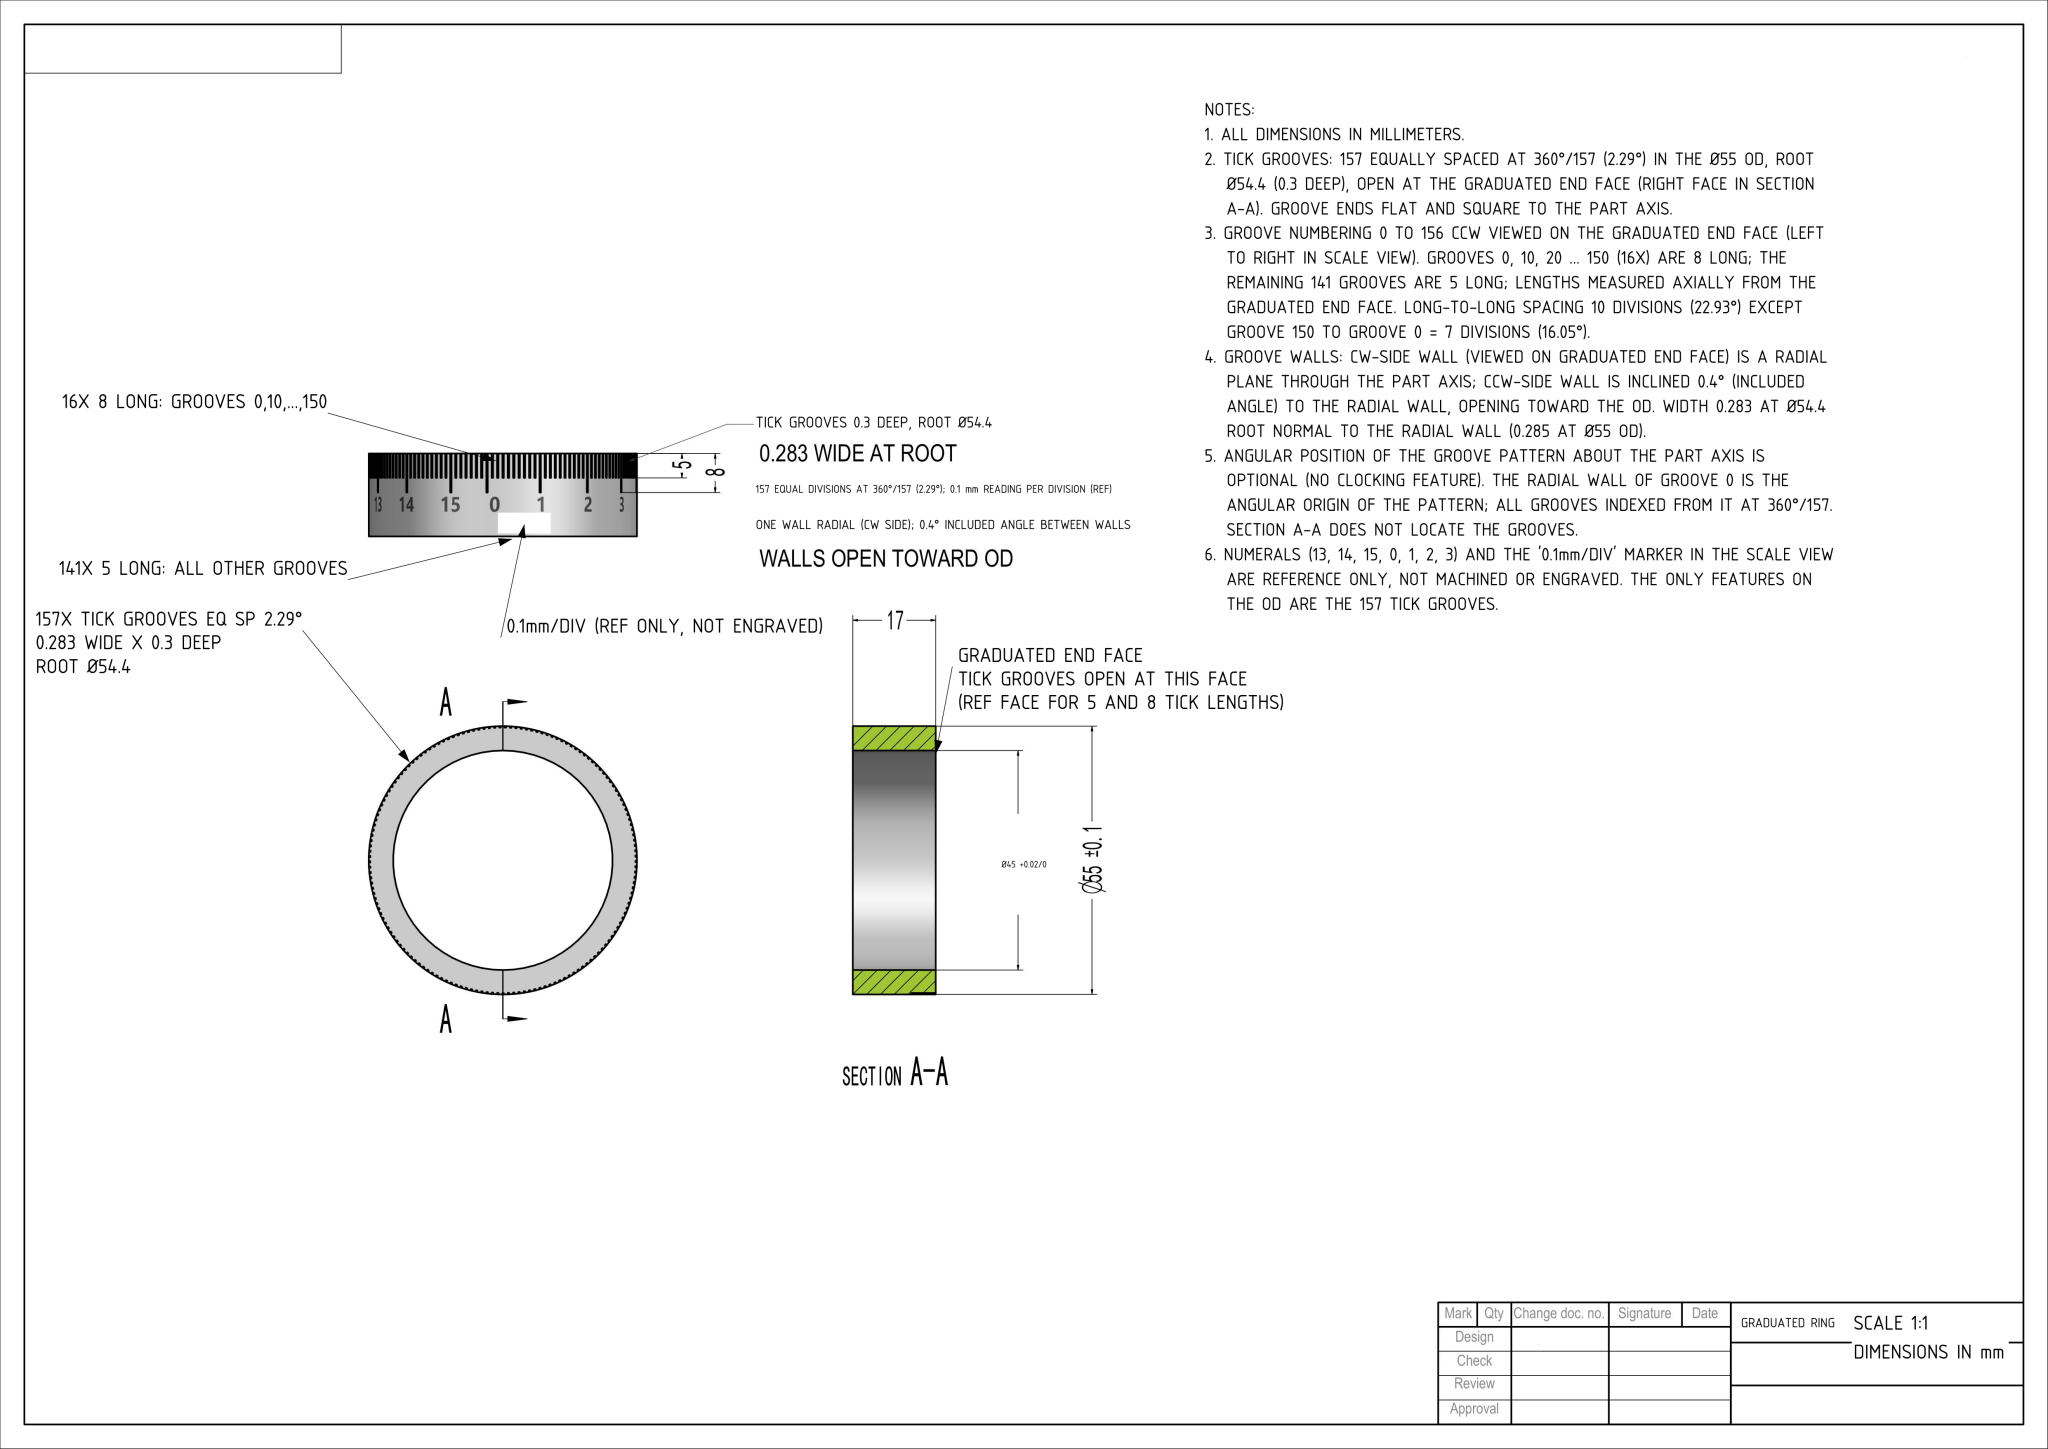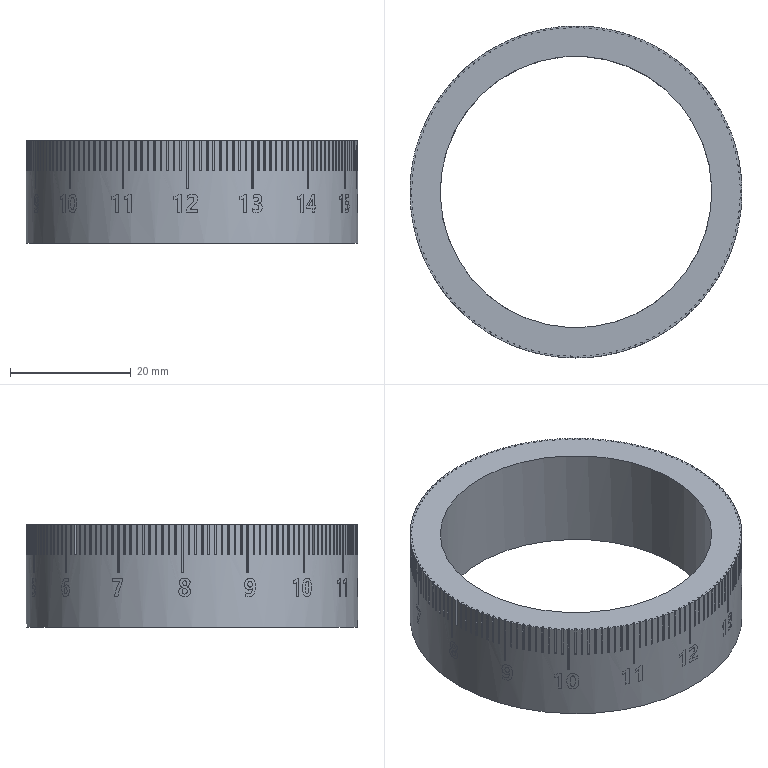Part | NX | mm | 1 solid | 672 faces | box 55 x 55 x 17 mm | volume 13282 mm3 | plane 473 | cylinder 199 | commonest cylinder face diameters 54.4 x157 55 x41 45 x1